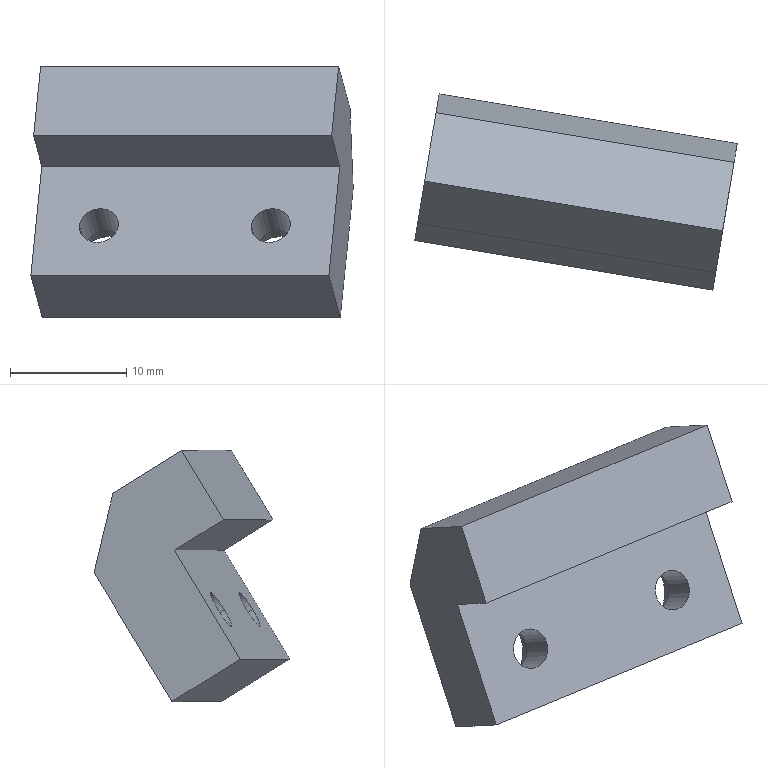Component | SolidWorks | 14AC-24-1-011-1 | 1 solid | 19 faces | box 27.74 x 16.86 x 21.62 mm | volume 3570 mm3 | plane 11 | cylinder 8 | commonest cylinder face diameters 6.5 x4 3.4 x4
build123d program:
from build123d import *

# Parameters (mm, degrees)
BOSS_EXTRUDE1_DEPTH                             = 11
BOSS_EXTRUDE1_DEPTH_BACK                        = 1
SKETCH1_W                                       = 26
SKETCH1_H                                       = 18
SKETCH2_W                                       = 26
SKETCH2_H                                       = 5
CUT_EXTRUDE1_DEPTH                              = 11
CHAMFER1_SIZE                                   = 5
M3_HEX_SOCKET_HEAD_CAP_SCREW_CBORE1_D           = 3.4
M3_HEX_SOCKET_HEAD_CAP_SCREW_CBORE1_CBORE_D     = 6.5
M3_HEX_SOCKET_HEAD_CAP_SCREW_CBORE1_CBORE_DEPTH = 3.4


with BuildPart() as part:
    # Sketch1 → Boss-Extrude1 (new, two sides: drawn at the far end of the back side and taken through both)
    with BuildSketch(Plane.XY.offset(-BOSS_EXTRUDE1_DEPTH_BACK)):
        Rectangle(SKETCH1_W, SKETCH1_H)
    extrude(amount=BOSS_EXTRUDE1_DEPTH + BOSS_EXTRUDE1_DEPTH_BACK)

    # Sketch2 → Cut-Extrude1 (cut)
    with BuildSketch(Plane(origin=(0, 9, 0), x_dir=(1, 0, 0), z_dir=(0, 1, 0))):
        with Locations((0, -8.5)):
            Rectangle(SKETCH2_W, SKETCH2_H)
    extrude(amount=-CUT_EXTRUDE1_DEPTH, mode=Mode.SUBTRACT)

    # Chamfer1
    chamfer1_edges = [part.edges().sort_by_distance(p)[0] for p in [
        (0, -9, -1),
    ]]
    chamfer(chamfer1_edges, length=CHAMFER1_SIZE)

    # M3 Hex Socket Head Cap Screw CBORE1 (through all)
    with Locations(Plane(origin=(-7.5, 4, -1), x_dir=(-1, 0, 0), z_dir=(0, 0, -1))):
        with Locations((0, 0), (-15, 0)):
            CounterBoreHole(M3_HEX_SOCKET_HEAD_CAP_SCREW_CBORE1_D / 2, M3_HEX_SOCKET_HEAD_CAP_SCREW_CBORE1_CBORE_D / 2, M3_HEX_SOCKET_HEAD_CAP_SCREW_CBORE1_CBORE_DEPTH)


solid = part.part

# Placed as in the assembly
solid = solid.moved(Location((524.43, -238.854, -65.033), (58.173, -8.052, 175.031)))
STEP:
#1=CARTESIAN_POINT('',(20.785,-9.592,-2.645));
#2=VERTEX_POINT('',#1);
#3=CARTESIAN_POINT('',(21.038,-9.634,-2.645));
#4=VERTEX_POINT('',#3);
#5=CARTESIAN_POINT('',(20.911,-9.613,-2.645));
#6=DIRECTION('',(0.1401,0.8413,-0.5222));
#7=DIRECTION('',(0.9864,-0.1642,0.));
#8=AXIS2_PLACEMENT_3D('',#5,#6,#7);
#9=CIRCLE('',#8,0.128);
#10=EDGE_CURVE('',#2,#4,#9,.T.);
#11=ORIENTED_EDGE('',*,*,#10,.F.);
#12=CARTESIAN_POINT('',(20.804,-9.479,-2.715));
#13=VERTEX_POINT('',#12);
#14=CARTESIAN_POINT('',(20.804,-9.479,-2.715));
#15=DIRECTION('',(0.1401,0.8413,-0.5222));
#16=VECTOR('',#15,39.37);
#17=LINE('',#14,#16);
#18=EDGE_CURVE('',#2,#13,#17,.T.);
#19=ORIENTED_EDGE('',*,*,#18,.T.);
#20=CARTESIAN_POINT('',(21.056,-9.521,-2.715));
#21=VERTEX_POINT('',#20);
#22=CARTESIAN_POINT('',(20.93,-9.5,-2.715));
#23=DIRECTION('',(0.1401,0.8413,-0.5222));
#24=DIRECTION('',(0.9864,-0.1642,0.));
#25=AXIS2_PLACEMENT_3D('',#22,#23,#24);
#26=CIRCLE('',#25,0.128);
#27=EDGE_CURVE('',#13,#21,#26,.T.);
#28=ORIENTED_EDGE('',*,*,#27,.T.);
#29=CARTESIAN_POINT('',(21.056,-9.521,-2.715));
#30=DIRECTION('',(0.1401,0.8413,-0.5222));
#31=VECTOR('',#30,39.37);
#32=LINE('',#29,#31);
#33=EDGE_CURVE('',#4,#21,#32,.T.);
#34=ORIENTED_EDGE('',*,*,#33,.F.);
#35=EDGE_LOOP('',(#11,#19,#28,#34));
#36=FACE_OUTER_BOUND('',#35,.T.);
#37=CARTESIAN_POINT('',(20.93,-9.5,-2.715));
#38=DIRECTION('',(0.1401,0.8413,-0.5222));
#39=DIRECTION('',(0.9864,-0.1642,0.));
#40=AXIS2_PLACEMENT_3D('',#37,#38,#39);
#41=CYLINDRICAL_SURFACE('',#40,0.128);
#42=ADVANCED_FACE('',(#36),#41,.F.);
#43=CARTESIAN_POINT('',(20.826,-9.721,-2.571));
#44=VERTEX_POINT('',#43);
#45=CARTESIAN_POINT('',(20.958,-9.743,-2.571));
#46=VERTEX_POINT('',#45);
#47=CARTESIAN_POINT('',(20.892,-9.732,-2.571));
#48=DIRECTION('',(0.1401,0.8413,-0.5222));
#49=DIRECTION('',(0.9864,-0.1642,0.));
#50=AXIS2_PLACEMENT_3D('',#47,#48,#49);
#51=CIRCLE('',#50,0.06693);
#52=EDGE_CURVE('',#44,#46,#51,.T.);
#53=ORIENTED_EDGE('',*,*,#52,.F.);
#54=CARTESIAN_POINT('',(20.845,-9.602,-2.645));
#55=VERTEX_POINT('',#54);
#56=CARTESIAN_POINT('',(20.864,-9.489,-2.715));
#57=DIRECTION('',(0.1401,0.8413,-0.5222));
#58=VECTOR('',#57,39.37);
#59=LINE('',#56,#58);
#60=EDGE_CURVE('',#44,#55,#59,.T.);
#61=ORIENTED_EDGE('',*,*,#60,.T.);
#62=CARTESIAN_POINT('',(20.977,-9.624,-2.645));
#63=VERTEX_POINT('',#62);
#64=CARTESIAN_POINT('',(20.911,-9.613,-2.645));
#65=DIRECTION('',(0.1401,0.8413,-0.5222));
#66=DIRECTION('',(0.9864,-0.1642,0.));
#67=AXIS2_PLACEMENT_3D('',#64,#65,#66);
#68=CIRCLE('',#67,0.06693);
#69=EDGE_CURVE('',#55,#63,#68,.T.);
#70=ORIENTED_EDGE('',*,*,#69,.T.);
#71=CARTESIAN_POINT('',(20.996,-9.511,-2.715));
#72=DIRECTION('',(0.1401,0.8413,-0.5222));
#73=VECTOR('',#72,39.37);
#74=LINE('',#71,#73);
#75=EDGE_CURVE('',#46,#63,#74,.T.);
#76=ORIENTED_EDGE('',*,*,#75,.F.);
#77=EDGE_LOOP('',(#53,#61,#70,#76));
#78=FACE_OUTER_BOUND('',#77,.T.);
#79=CARTESIAN_POINT('',(20.93,-9.5,-2.715));
#80=DIRECTION('',(0.1401,0.8413,-0.5222));
#81=DIRECTION('',(0.9864,-0.1642,0.));
#82=AXIS2_PLACEMENT_3D('',#79,#80,#81);
#83=CYLINDRICAL_SURFACE('',#82,0.06693);
#84=ADVANCED_FACE('',(#78),#83,.F.);
#85=CARTESIAN_POINT('',(20.203,-9.495,-2.645));
#86=VERTEX_POINT('',#85);
#87=CARTESIAN_POINT('',(20.455,-9.537,-2.645));
#88=VERTEX_POINT('',#87);
#89=CARTESIAN_POINT('',(20.329,-9.516,-2.645));
#90=DIRECTION('',(0.1401,0.8413,-0.5222));
#91=DIRECTION('',(0.9864,-0.1642,0.));
#92=AXIS2_PLACEMENT_3D('',#89,#90,#91);
#93=CIRCLE('',#92,0.128);
#94=EDGE_CURVE('',#86,#88,#93,.T.);
#95=ORIENTED_EDGE('',*,*,#94,.F.);
#96=CARTESIAN_POINT('',(20.221,-9.382,-2.715));
#97=VERTEX_POINT('',#96);
#98=CARTESIAN_POINT('',(20.221,-9.382,-2.715));
#99=DIRECTION('',(0.1401,0.8413,-0.5222));
#100=VECTOR('',#99,39.37);
#101=LINE('',#98,#100);
#102=EDGE_CURVE('',#86,#97,#101,.T.);
#103=ORIENTED_EDGE('',*,*,#102,.T.);
#104=CARTESIAN_POINT('',(20.474,-9.424,-2.715));
#105=VERTEX_POINT('',#104);
#106=CARTESIAN_POINT('',(20.348,-9.403,-2.715));
#107=DIRECTION('',(0.1401,0.8413,-0.5222));
#108=DIRECTION('',(0.9864,-0.1642,0.));
#109=AXIS2_PLACEMENT_3D('',#106,#107,#108);
#110=CIRCLE('',#109,0.128);
#111=EDGE_CURVE('',#97,#105,#110,.T.);
#112=ORIENTED_EDGE('',*,*,#111,.T.);
#113=CARTESIAN_POINT('',(20.474,-9.424,-2.715));
#114=DIRECTION('',(0.1401,0.8413,-0.5222));
#115=VECTOR('',#114,39.37);
#116=LINE('',#113,#115);
#117=EDGE_CURVE('',#88,#105,#116,.T.);
#118=ORIENTED_EDGE('',*,*,#117,.F.);
#119=EDGE_LOOP('',(#95,#103,#112,#118));
#120=FACE_OUTER_BOUND('',#119,.T.);
#121=CARTESIAN_POINT('',(20.348,-9.403,-2.715));
#122=DIRECTION('',(0.1401,0.8413,-0.5222));
#123=DIRECTION('',(0.9864,-0.1642,0.));
#124=AXIS2_PLACEMENT_3D('',#121,#122,#123);
#125=CYLINDRICAL_SURFACE('',#124,0.128);
#126=ADVANCED_FACE('',(#120),#125,.F.);
#127=CARTESIAN_POINT('',(20.243,-9.624,-2.571));
#128=VERTEX_POINT('',#127);
#129=CARTESIAN_POINT('',(20.375,-9.646,-2.571));
#130=VERTEX_POINT('',#129);
#131=CARTESIAN_POINT('',(20.309,-9.635,-2.571));
#132=DIRECTION('',(0.1401,0.8413,-0.5222));
#133=DIRECTION('',(0.9864,-0.1642,0.));
#134=AXIS2_PLACEMENT_3D('',#131,#132,#133);
#135=CIRCLE('',#134,0.06693);
#136=EDGE_CURVE('',#128,#130,#135,.T.);
#137=ORIENTED_EDGE('',*,*,#136,.F.);
#138=CARTESIAN_POINT('',(20.263,-9.505,-2.645));
#139=VERTEX_POINT('',#138);
#140=CARTESIAN_POINT('',(20.282,-9.392,-2.715));
#141=DIRECTION('',(0.1401,0.8413,-0.5222));
#142=VECTOR('',#141,39.37);
#143=LINE('',#140,#142);
#144=EDGE_CURVE('',#128,#139,#143,.T.);
#145=ORIENTED_EDGE('',*,*,#144,.T.);
#146=CARTESIAN_POINT('',(20.395,-9.527,-2.645));
#147=VERTEX_POINT('',#146);
#148=CARTESIAN_POINT('',(20.329,-9.516,-2.645));
#149=DIRECTION('',(0.1401,0.8413,-0.5222));
#150=DIRECTION('',(0.9864,-0.1642,0.));
#151=AXIS2_PLACEMENT_3D('',#148,#149,#150);
#152=CIRCLE('',#151,0.06693);
#153=EDGE_CURVE('',#139,#147,#152,.T.);
#154=ORIENTED_EDGE('',*,*,#153,.T.);
#155=CARTESIAN_POINT('',(20.414,-9.414,-2.715));
#156=DIRECTION('',(0.1401,0.8413,-0.5222));
#157=VECTOR('',#156,39.37);
#158=LINE('',#155,#157);
#159=EDGE_CURVE('',#130,#147,#158,.T.);
#160=ORIENTED_EDGE('',*,*,#159,.F.);
#161=EDGE_LOOP('',(#137,#145,#154,#160));
#162=FACE_OUTER_BOUND('',#161,.T.);
#163=CARTESIAN_POINT('',(20.348,-9.403,-2.715));
#164=DIRECTION('',(0.1401,0.8413,-0.5222));
#165=DIRECTION('',(0.9864,-0.1642,0.));
#166=AXIS2_PLACEMENT_3D('',#163,#164,#165);
#167=CYLINDRICAL_SURFACE('',#166,0.06693);
#168=ADVANCED_FACE('',(#162),#167,.F.);
#169=CARTESIAN_POINT('',(20.112,-9.501,-2.032));
#170=VERTEX_POINT('',#169);
#171=CARTESIAN_POINT('',(20.088,-9.643,-2.267));
#172=VERTEX_POINT('',#171);
#173=CARTESIAN_POINT('',(20.051,-9.866,-2.636));
#174=DIRECTION('',(-0.08576,-0.5151,-0.8529));
#175=VECTOR('',#174,39.37);
#176=LINE('',#173,#175);
#177=EDGE_CURVE('',#170,#172,#176,.T.);
#178=ORIENTED_EDGE('',*,*,#177,.T.);
#179=CARTESIAN_POINT('',(21.098,-9.812,-2.267));
#180=VERTEX_POINT('',#179);
#181=CARTESIAN_POINT('',(20.088,-9.643,-2.267));
#182=DIRECTION('',(-0.9864,0.1642,-0.));
#183=VECTOR('',#182,39.37);
#184=LINE('',#181,#183);
#185=EDGE_CURVE('',#180,#172,#184,.T.);
#186=ORIENTED_EDGE('',*,*,#185,.F.);
#187=CARTESIAN_POINT('',(21.121,-9.67,-2.032));
#188=VERTEX_POINT('',#187);
#189=CARTESIAN_POINT('',(21.061,-10.035,-2.636));
#190=DIRECTION('',(0.08576,0.5151,0.8529));
#191=VECTOR('',#190,39.37);
#192=LINE('',#189,#191);
#193=EDGE_CURVE('',#180,#188,#192,.T.);
#194=ORIENTED_EDGE('',*,*,#193,.T.);
#195=CARTESIAN_POINT('',(21.121,-9.67,-2.032));
#196=DIRECTION('',(-0.9864,0.1642,-0.));
#197=VECTOR('',#196,39.37);
#198=LINE('',#195,#197);
#199=EDGE_CURVE('',#188,#170,#198,.T.);
#200=ORIENTED_EDGE('',*,*,#199,.T.);
#201=EDGE_LOOP('',(#178,#186,#194,#200));
#202=FACE_OUTER_BOUND('',#201,.T.);
#203=CARTESIAN_POINT('',(20.586,-9.768,-2.334));
#204=DIRECTION('',(-0.1401,-0.8413,0.5222));
#205=DIRECTION('',(-0.9864,0.1642,-0.));
#206=AXIS2_PLACEMENT_3D('',#203,#204,#205);
#207=PLANE('',#206);
#208=ADVANCED_FACE('',(#202),#207,.T.);
#209=CARTESIAN_POINT('',(20.15,-9.27,-2.176));
#210=VERTEX_POINT('',#209);
#211=CARTESIAN_POINT('',(20.178,-9.104,-2.279));
#212=DIRECTION('',(-0.1401,-0.8413,0.5222));
#213=VECTOR('',#212,39.37);
#214=LINE('',#211,#213);
#215=EDGE_CURVE('',#210,#170,#214,.T.);
#216=ORIENTED_EDGE('',*,*,#215,.F.);
#217=CARTESIAN_POINT('',(20.161,-9.205,-2.447));
#218=VERTEX_POINT('',#217);
#219=CARTESIAN_POINT('',(20.175,-9.122,-2.798));
#220=DIRECTION('',(0.03841,0.2307,-0.9723));
#221=VECTOR('',#220,39.37);
#222=LINE('',#219,#221);
#223=EDGE_CURVE('',#210,#218,#222,.T.);
#224=ORIENTED_EDGE('',*,*,#223,.T.);
#225=CARTESIAN_POINT('',(20.117,-9.469,-2.883));
#226=VERTEX_POINT('',#225);
#227=CARTESIAN_POINT('',(20.117,-9.469,-2.883));
#228=DIRECTION('',(-0.08576,-0.5151,-0.8529));
#229=VECTOR('',#228,39.37);
#230=LINE('',#227,#229);
#231=EDGE_CURVE('',#218,#226,#230,.T.);
#232=ORIENTED_EDGE('',*,*,#231,.T.);
#233=CARTESIAN_POINT('',(20.079,-9.701,-2.739));
#234=VERTEX_POINT('',#233);
#235=CARTESIAN_POINT('',(20.117,-9.469,-2.883));
#236=DIRECTION('',(-0.1401,-0.8413,0.5222));
#237=VECTOR('',#236,39.37);
#238=LINE('',#235,#237);
#239=EDGE_CURVE('',#226,#234,#238,.T.);
#240=ORIENTED_EDGE('',*,*,#239,.T.);
#241=CARTESIAN_POINT('',(20.116,-9.478,-2.37));
#242=VERTEX_POINT('',#241);
#243=CARTESIAN_POINT('',(20.116,-9.478,-2.37));
#244=DIRECTION('',(-0.08576,-0.5151,-0.8529));
#245=VECTOR('',#244,39.37);
#246=LINE('',#243,#245);
#247=EDGE_CURVE('',#242,#234,#246,.T.);
#248=ORIENTED_EDGE('',*,*,#247,.F.);
#249=CARTESIAN_POINT('',(20.088,-9.643,-2.267));
#250=DIRECTION('',(0.1401,0.8413,-0.5222));
#251=VECTOR('',#250,39.37);
#252=LINE('',#249,#251);
#253=EDGE_CURVE('',#172,#242,#252,.T.);
#254=ORIENTED_EDGE('',*,*,#253,.F.);
#255=ORIENTED_EDGE('',*,*,#177,.F.);
#256=EDGE_LOOP('',(#216,#224,#232,#240,#248,#254,#255));
#257=FACE_OUTER_BOUND('',#256,.T.);
#258=CARTESIAN_POINT('',(20.117,-9.469,-2.883));
#259=DIRECTION('',(-0.9864,0.1642,-0.));
#260=DIRECTION('',(-0.08576,-0.5151,-0.8529));
#261=AXIS2_PLACEMENT_3D('',#258,#259,#260);
#262=PLANE('',#261);
#263=ADVANCED_FACE('',(#257),#262,.T.);
#264=CARTESIAN_POINT('',(21.16,-9.438,-2.176));
#265=VERTEX_POINT('',#264);
#266=CARTESIAN_POINT('',(21.188,-9.272,-2.279));
#267=DIRECTION('',(-0.1401,-0.8413,0.5222));
#268=VECTOR('',#267,39.37);
#269=LINE('',#266,#268);
#270=EDGE_CURVE('',#265,#188,#269,.T.);
#271=ORIENTED_EDGE('',*,*,#270,.F.);
#272=CARTESIAN_POINT('',(20.15,-9.27,-2.176));
#273=DIRECTION('',(-0.9864,0.1642,-0.));
#274=VECTOR('',#273,39.37);
#275=LINE('',#272,#274);
#276=EDGE_CURVE('',#265,#210,#275,.T.);
#277=ORIENTED_EDGE('',*,*,#276,.T.);
#278=ORIENTED_EDGE('',*,*,#215,.T.);
#279=ORIENTED_EDGE('',*,*,#199,.F.);
#280=EDGE_LOOP('',(#271,#277,#278,#279));
#281=FACE_OUTER_BOUND('',#280,.T.);
#282=CARTESIAN_POINT('',(21.188,-9.272,-2.279));
#283=DIRECTION('',(0.08576,0.5151,0.8529));
#284=DIRECTION('',(0.1401,0.8413,-0.5222));
#285=AXIS2_PLACEMENT_3D('',#282,#283,#284);
#286=PLANE('',#285);
#287=ADVANCED_FACE('',(#281),#286,.T.);
#288=CARTESIAN_POINT('',(21.127,-9.637,-2.883));
#289=VERTEX_POINT('',#288);
#290=CARTESIAN_POINT('',(21.171,-9.374,-2.447));
#291=VERTEX_POINT('',#290);
#292=CARTESIAN_POINT('',(21.127,-9.637,-2.883));
#293=DIRECTION('',(0.08576,0.5151,0.8529));
#294=VECTOR('',#293,39.37);
#295=LINE('',#292,#294);
#296=EDGE_CURVE('',#289,#291,#295,.T.);
#297=ORIENTED_EDGE('',*,*,#296,.T.);
#298=CARTESIAN_POINT('',(21.185,-9.29,-2.798));
#299=DIRECTION('',(-0.03841,-0.2307,0.9723));
#300=VECTOR('',#299,39.37);
#301=LINE('',#298,#300);
#302=EDGE_CURVE('',#291,#265,#301,.T.);
#303=ORIENTED_EDGE('',*,*,#302,.T.);
#304=ORIENTED_EDGE('',*,*,#270,.T.);
#305=ORIENTED_EDGE('',*,*,#193,.F.);
#306=CARTESIAN_POINT('',(21.125,-9.646,-2.37));
#307=VERTEX_POINT('',#306);
#308=CARTESIAN_POINT('',(21.098,-9.812,-2.267));
#309=DIRECTION('',(-0.1401,-0.8413,0.5222));
#310=VECTOR('',#309,39.37);
#311=LINE('',#308,#310);
#312=EDGE_CURVE('',#307,#180,#311,.T.);
#313=ORIENTED_EDGE('',*,*,#312,.F.);
#314=CARTESIAN_POINT('',(21.088,-9.869,-2.739));
#315=VERTEX_POINT('',#314);
#316=CARTESIAN_POINT('',(21.125,-9.646,-2.37));
#317=DIRECTION('',(-0.08576,-0.5151,-0.8529));
#318=VECTOR('',#317,39.37);
#319=LINE('',#316,#318);
#320=EDGE_CURVE('',#307,#315,#319,.T.);
#321=ORIENTED_EDGE('',*,*,#320,.T.);
#322=CARTESIAN_POINT('',(21.127,-9.637,-2.883));
#323=DIRECTION('',(-0.1401,-0.8413,0.5222));
#324=VECTOR('',#323,39.37);
#325=LINE('',#322,#324);
#326=EDGE_CURVE('',#289,#315,#325,.T.);
#327=ORIENTED_EDGE('',*,*,#326,.F.);
#328=EDGE_LOOP('',(#297,#303,#304,#305,#313,#321,#327));
#329=FACE_OUTER_BOUND('',#328,.T.);
#330=CARTESIAN_POINT('',(21.127,-9.637,-2.883));
#331=DIRECTION('',(0.9864,-0.1642,0.));
#332=DIRECTION('',(0.08576,0.5151,0.8529));
#333=AXIS2_PLACEMENT_3D('',#330,#331,#332);
#334=PLANE('',#333);
#335=ADVANCED_FACE('',(#329),#334,.T.);
#336=CARTESIAN_POINT('',(20.079,-9.701,-2.739));
#337=DIRECTION('',(0.9864,-0.1642,0.));
#338=VECTOR('',#337,39.37);
#339=LINE('',#336,#338);
#340=EDGE_CURVE('',#234,#315,#339,.T.);
#341=ORIENTED_EDGE('',*,*,#340,.F.);
#342=ORIENTED_EDGE('',*,*,#239,.F.);
#343=CARTESIAN_POINT('',(21.127,-9.637,-2.883));
#344=DIRECTION('',(0.9864,-0.1642,0.));
#345=VECTOR('',#344,39.37);
#346=LINE('',#343,#345);
#347=EDGE_CURVE('',#226,#289,#346,.T.);
#348=ORIENTED_EDGE('',*,*,#347,.T.);
#349=ORIENTED_EDGE('',*,*,#326,.T.);
#350=EDGE_LOOP('',(#341,#342,#348,#349));
#351=FACE_OUTER_BOUND('',#350,.T.);
#352=CARTESIAN_POINT('',(21.127,-9.637,-2.883));
#353=DIRECTION('',(-0.08576,-0.5151,-0.8529));
#354=DIRECTION('',(-0.1401,-0.8413,0.5222));
#355=AXIS2_PLACEMENT_3D('',#352,#353,#354);
#356=PLANE('',#355);
#357=ADVANCED_FACE('',(#351),#356,.T.);
#358=CARTESIAN_POINT('',(20.93,-9.5,-2.715));
#359=DIRECTION('',(0.1401,0.8413,-0.5222));
#360=DIRECTION('',(0.9864,-0.1642,0.));
#361=AXIS2_PLACEMENT_3D('',#358,#359,#360);
#362=CIRCLE('',#361,0.128);
#363=EDGE_CURVE('',#21,#13,#362,.T.);
#364=ORIENTED_EDGE('',*,*,#363,.F.);
#365=ORIENTED_EDGE('',*,*,#27,.F.);
#366=EDGE_LOOP('',(#364,#365));
#367=FACE_BOUND('',#366,.T.);
#368=CARTESIAN_POINT('',(20.348,-9.403,-2.715));
#369=DIRECTION('',(0.1401,0.8413,-0.5222));
#370=DIRECTION('',(0.9864,-0.1642,0.));
#371=AXIS2_PLACEMENT_3D('',#368,#369,#370);
#372=CIRCLE('',#371,0.128);
#373=EDGE_CURVE('',#105,#97,#372,.T.);
#374=ORIENTED_EDGE('',*,*,#373,.F.);
#375=ORIENTED_EDGE('',*,*,#111,.F.);
#376=EDGE_LOOP('',(#374,#375));
#377=FACE_BOUND('',#376,.T.);
#378=ORIENTED_EDGE('',*,*,#231,.F.);
#379=CARTESIAN_POINT('',(21.171,-9.374,-2.447));
#380=DIRECTION('',(0.9864,-0.1642,0.));
#381=VECTOR('',#380,39.37);
#382=LINE('',#379,#381);
#383=EDGE_CURVE('',#218,#291,#382,.T.);
#384=ORIENTED_EDGE('',*,*,#383,.T.);
#385=ORIENTED_EDGE('',*,*,#296,.F.);
#386=ORIENTED_EDGE('',*,*,#347,.F.);
#387=EDGE_LOOP('',(#378,#384,#385,#386));
#388=FACE_OUTER_BOUND('',#387,.T.);
#389=CARTESIAN_POINT('',(20.652,-9.371,-2.581));
#390=DIRECTION('',(-0.1401,-0.8413,0.5222));
#391=DIRECTION('',(-0.9864,0.1642,-0.));
#392=AXIS2_PLACEMENT_3D('',#389,#390,#391);
#393=PLANE('',#392);
#394=ADVANCED_FACE('',(#367,#377,#388),#393,.F.);
#395=CARTESIAN_POINT('',(20.892,-9.732,-2.571));
#396=DIRECTION('',(0.1401,0.8413,-0.5222));
#397=DIRECTION('',(0.9864,-0.1642,0.));
#398=AXIS2_PLACEMENT_3D('',#395,#396,#397);
#399=CIRCLE('',#398,0.06693);
#400=EDGE_CURVE('',#46,#44,#399,.T.);
#401=ORIENTED_EDGE('',*,*,#400,.T.);
#402=ORIENTED_EDGE('',*,*,#52,.T.);
#403=EDGE_LOOP('',(#401,#402));
#404=FACE_BOUND('',#403,.T.);
#405=CARTESIAN_POINT('',(20.309,-9.635,-2.571));
#406=DIRECTION('',(0.1401,0.8413,-0.5222));
#407=DIRECTION('',(0.9864,-0.1642,0.));
#408=AXIS2_PLACEMENT_3D('',#405,#406,#407);
#409=CIRCLE('',#408,0.06693);
#410=EDGE_CURVE('',#130,#128,#409,.T.);
#411=ORIENTED_EDGE('',*,*,#410,.T.);
#412=ORIENTED_EDGE('',*,*,#136,.T.);
#413=EDGE_LOOP('',(#411,#412));
#414=FACE_BOUND('',#413,.T.);
#415=ORIENTED_EDGE('',*,*,#340,.T.);
#416=ORIENTED_EDGE('',*,*,#320,.F.);
#417=CARTESIAN_POINT('',(20.116,-9.478,-2.37));
#418=DIRECTION('',(0.9864,-0.1642,0.));
#419=VECTOR('',#418,39.37);
#420=LINE('',#417,#419);
#421=EDGE_CURVE('',#242,#307,#420,.T.);
#422=ORIENTED_EDGE('',*,*,#421,.F.);
#423=ORIENTED_EDGE('',*,*,#247,.T.);
#424=EDGE_LOOP('',(#415,#416,#422,#423));
#425=FACE_OUTER_BOUND('',#424,.T.);
#426=CARTESIAN_POINT('',(20.116,-9.478,-2.37));
#427=DIRECTION('',(0.1401,0.8413,-0.5222));
#428=DIRECTION('',(0.9864,-0.1642,0.));
#429=AXIS2_PLACEMENT_3D('',#426,#427,#428);
#430=PLANE('',#429);
#431=ADVANCED_FACE('',(#404,#414,#425),#430,.F.);
#432=ORIENTED_EDGE('',*,*,#253,.T.);
#433=ORIENTED_EDGE('',*,*,#421,.T.);
#434=ORIENTED_EDGE('',*,*,#312,.T.);
#435=ORIENTED_EDGE('',*,*,#185,.T.);
#436=EDGE_LOOP('',(#432,#433,#434,#435));
#437=FACE_OUTER_BOUND('',#436,.T.);
#438=CARTESIAN_POINT('',(20.654,-9.363,-2.493));
#439=DIRECTION('',(-0.08576,-0.5151,-0.8529));
#440=DIRECTION('',(-0.1401,-0.8413,0.5222));
#441=AXIS2_PLACEMENT_3D('',#438,#439,#440);
#442=PLANE('',#441);
#443=ADVANCED_FACE('',(#437),#442,.T.);
#444=ORIENTED_EDGE('',*,*,#302,.F.);
#445=ORIENTED_EDGE('',*,*,#383,.F.);
#446=ORIENTED_EDGE('',*,*,#223,.F.);
#447=ORIENTED_EDGE('',*,*,#276,.F.);
#448=EDGE_LOOP('',(#444,#445,#446,#447));
#449=FACE_OUTER_BOUND('',#448,.T.);
#450=CARTESIAN_POINT('',(21.16,-9.438,-2.176));
#451=DIRECTION('',(0.1597,0.9591,0.2338));
#452=DIRECTION('',(0.9864,-0.1642,0.));
#453=AXIS2_PLACEMENT_3D('',#450,#451,#452);
#454=PLANE('',#453);
#455=ADVANCED_FACE('',(#449),#454,.T.);
#456=ORIENTED_EDGE('',*,*,#144,.F.);
#457=ORIENTED_EDGE('',*,*,#410,.F.);
#458=ORIENTED_EDGE('',*,*,#159,.T.);
#459=CARTESIAN_POINT('',(20.329,-9.516,-2.645));
#460=DIRECTION('',(0.1401,0.8413,-0.5222));
#461=DIRECTION('',(0.9864,-0.1642,0.));
#462=AXIS2_PLACEMENT_3D('',#459,#460,#461);
#463=CIRCLE('',#462,0.06693);
#464=EDGE_CURVE('',#147,#139,#463,.T.);
#465=ORIENTED_EDGE('',*,*,#464,.T.);
#466=EDGE_LOOP('',(#456,#457,#458,#465));
#467=FACE_OUTER_BOUND('',#466,.T.);
#468=CARTESIAN_POINT('',(20.348,-9.403,-2.715));
#469=DIRECTION('',(0.1401,0.8413,-0.5222));
#470=DIRECTION('',(0.9864,-0.1642,0.));
#471=AXIS2_PLACEMENT_3D('',#468,#469,#470);
#472=CYLINDRICAL_SURFACE('',#471,0.06693);
#473=ADVANCED_FACE('',(#467),#472,.F.);
#474=ORIENTED_EDGE('',*,*,#464,.F.);
#475=ORIENTED_EDGE('',*,*,#153,.F.);
#476=EDGE_LOOP('',(#474,#475));
#477=FACE_BOUND('',#476,.T.);
#478=CARTESIAN_POINT('',(20.329,-9.516,-2.645));
#479=DIRECTION('',(0.1401,0.8413,-0.5222));
#480=DIRECTION('',(0.9864,-0.1642,0.));
#481=AXIS2_PLACEMENT_3D('',#478,#479,#480);
#482=CIRCLE('',#481,0.128);
#483=EDGE_CURVE('',#88,#86,#482,.T.);
#484=ORIENTED_EDGE('',*,*,#483,.T.);
#485=ORIENTED_EDGE('',*,*,#94,.T.);
#486=EDGE_LOOP('',(#484,#485));
#487=FACE_OUTER_BOUND('',#486,.T.);
#488=CARTESIAN_POINT('',(20.263,-9.505,-2.645));
#489=DIRECTION('',(-0.1401,-0.8413,0.5222));
#490=DIRECTION('',(-0.9864,0.1642,-0.));
#491=AXIS2_PLACEMENT_3D('',#488,#489,#490);
#492=PLANE('',#491);
#493=ADVANCED_FACE('',(#477,#487),#492,.F.);
#494=ORIENTED_EDGE('',*,*,#102,.F.);
#495=ORIENTED_EDGE('',*,*,#483,.F.);
#496=ORIENTED_EDGE('',*,*,#117,.T.);
#497=ORIENTED_EDGE('',*,*,#373,.T.);
#498=EDGE_LOOP('',(#494,#495,#496,#497));
#499=FACE_OUTER_BOUND('',#498,.T.);
#500=CARTESIAN_POINT('',(20.348,-9.403,-2.715));
#501=DIRECTION('',(0.1401,0.8413,-0.5222));
#502=DIRECTION('',(0.9864,-0.1642,0.));
#503=AXIS2_PLACEMENT_3D('',#500,#501,#502);
#504=CYLINDRICAL_SURFACE('',#503,0.128);
#505=ADVANCED_FACE('',(#499),#504,.F.);
#506=ORIENTED_EDGE('',*,*,#60,.F.);
#507=ORIENTED_EDGE('',*,*,#400,.F.);
#508=ORIENTED_EDGE('',*,*,#75,.T.);
#509=CARTESIAN_POINT('',(20.911,-9.613,-2.645));
#510=DIRECTION('',(0.1401,0.8413,-0.5222));
#511=DIRECTION('',(0.9864,-0.1642,0.));
#512=AXIS2_PLACEMENT_3D('',#509,#510,#511);
#513=CIRCLE('',#512,0.06693);
#514=EDGE_CURVE('',#63,#55,#513,.T.);
#515=ORIENTED_EDGE('',*,*,#514,.T.);
#516=EDGE_LOOP('',(#506,#507,#508,#515));
#517=FACE_OUTER_BOUND('',#516,.T.);
#518=CARTESIAN_POINT('',(20.93,-9.5,-2.715));
#519=DIRECTION('',(0.1401,0.8413,-0.5222));
#520=DIRECTION('',(0.9864,-0.1642,0.));
#521=AXIS2_PLACEMENT_3D('',#518,#519,#520);
#522=CYLINDRICAL_SURFACE('',#521,0.06693);
#523=ADVANCED_FACE('',(#517),#522,.F.);
#524=ORIENTED_EDGE('',*,*,#514,.F.);
#525=ORIENTED_EDGE('',*,*,#69,.F.);
#526=EDGE_LOOP('',(#524,#525));
#527=FACE_BOUND('',#526,.T.);
#528=CARTESIAN_POINT('',(20.911,-9.613,-2.645));
#529=DIRECTION('',(0.1401,0.8413,-0.5222));
#530=DIRECTION('',(0.9864,-0.1642,0.));
#531=AXIS2_PLACEMENT_3D('',#528,#529,#530);
#532=CIRCLE('',#531,0.128);
#533=EDGE_CURVE('',#4,#2,#532,.T.);
#534=ORIENTED_EDGE('',*,*,#533,.T.);
#535=ORIENTED_EDGE('',*,*,#10,.T.);
#536=EDGE_LOOP('',(#534,#535));
#537=FACE_OUTER_BOUND('',#536,.T.);
#538=CARTESIAN_POINT('',(20.845,-9.602,-2.645));
#539=DIRECTION('',(-0.1401,-0.8413,0.5222));
#540=DIRECTION('',(-0.9864,0.1642,-0.));
#541=AXIS2_PLACEMENT_3D('',#538,#539,#540);
#542=PLANE('',#541);
#543=ADVANCED_FACE('',(#527,#537),#542,.F.);
#544=ORIENTED_EDGE('',*,*,#18,.F.);
#545=ORIENTED_EDGE('',*,*,#533,.F.);
#546=ORIENTED_EDGE('',*,*,#33,.T.);
#547=ORIENTED_EDGE('',*,*,#363,.T.);
#548=EDGE_LOOP('',(#544,#545,#546,#547));
#549=FACE_OUTER_BOUND('',#548,.T.);
#550=CARTESIAN_POINT('',(20.93,-9.5,-2.715));
#551=DIRECTION('',(0.1401,0.8413,-0.5222));
#552=DIRECTION('',(0.9864,-0.1642,0.));
#553=AXIS2_PLACEMENT_3D('',#550,#551,#552);
#554=CYLINDRICAL_SURFACE('',#553,0.128);
#555=ADVANCED_FACE('',(#549),#554,.F.);
#556=CLOSED_SHELL('',(#42,#84,#126,#168,#208,#263,#287,#335,#357,#394,#431,#443,#455,#473,#493,#505,#523,#543,#555));
#557=MANIFOLD_SOLID_BREP('',#556);
#558=CARTESIAN_POINT('',(0.,0.,0.));
#559=DIRECTION('',(0.,0.,1.));
#560=DIRECTION('',(1.,0.,0.));
#561=AXIS2_PLACEMENT_3D('',#558,#559,#560);
#562=(LENGTH_UNIT()NAMED_UNIT(*)SI_UNIT($,.METRE.));
#563=LENGTH_MEASURE_WITH_UNIT(LENGTH_MEASURE(0.0254),#562);
#564=DIMENSIONAL_EXPONENTS(1.,0.,0.,0.,0.,0.,0.);
#565=(CONVERSION_BASED_UNIT('',#563)LENGTH_UNIT()NAMED_UNIT(#564));
#566=UNCERTAINTY_MEASURE_WITH_UNIT(LENGTH_MEASURE(0.00001),#565,'','');
#567=(NAMED_UNIT(*)PLANE_ANGLE_UNIT()SI_UNIT($,.RADIAN.));
#568=(NAMED_UNIT(*)SI_UNIT($,.STERADIAN.)SOLID_ANGLE_UNIT());
#569=(GEOMETRIC_REPRESENTATION_CONTEXT(3)GLOBAL_UNCERTAINTY_ASSIGNED_CONTEXT((#566))GLOBAL_UNIT_ASSIGNED_CONTEXT((#565,#567,#568))REPRESENTATION_CONTEXT('',''));
#570=ADVANCED_BREP_SHAPE_REPRESENTATION('',(#557,#561),#569);
#571=COLOUR_RGB('',0.7922,0.8196,0.9333);
#572=FILL_AREA_STYLE_COLOUR('',#571);
#573=FILL_AREA_STYLE('',(#572));
#574=SURFACE_STYLE_FILL_AREA(#573);
#575=SURFACE_SIDE_STYLE('',(#574));
#576=SURFACE_STYLE_USAGE(.BOTH.,#575);
#577=PRESENTATION_STYLE_ASSIGNMENT((#576));
#578=STYLED_ITEM('',(#577),#557);
#579=(LENGTH_UNIT()NAMED_UNIT(*)SI_UNIT($,.METRE.));
#580=LENGTH_MEASURE_WITH_UNIT(LENGTH_MEASURE(0.0254),#579);
#581=DIMENSIONAL_EXPONENTS(1.,0.,0.,0.,0.,0.,0.);
#582=(CONVERSION_BASED_UNIT('',#580)LENGTH_UNIT()NAMED_UNIT(#581));
#583=UNCERTAINTY_MEASURE_WITH_UNIT(LENGTH_MEASURE(0.00001),#582,'','');
#584=(NAMED_UNIT(*)PLANE_ANGLE_UNIT()SI_UNIT($,.RADIAN.));
#585=(NAMED_UNIT(*)SI_UNIT($,.STERADIAN.)SOLID_ANGLE_UNIT());
#586=(GEOMETRIC_REPRESENTATION_CONTEXT(3)GLOBAL_UNCERTAINTY_ASSIGNED_CONTEXT((#583))GLOBAL_UNIT_ASSIGNED_CONTEXT((#582,#584,#585))REPRESENTATION_CONTEXT('',''));
#587=MECHANICAL_DESIGN_GEOMETRIC_PRESENTATION_REPRESENTATION('',(#578),#586);
#588=PRESENTATION_LAYER_ASSIGNMENT('','',(#578));